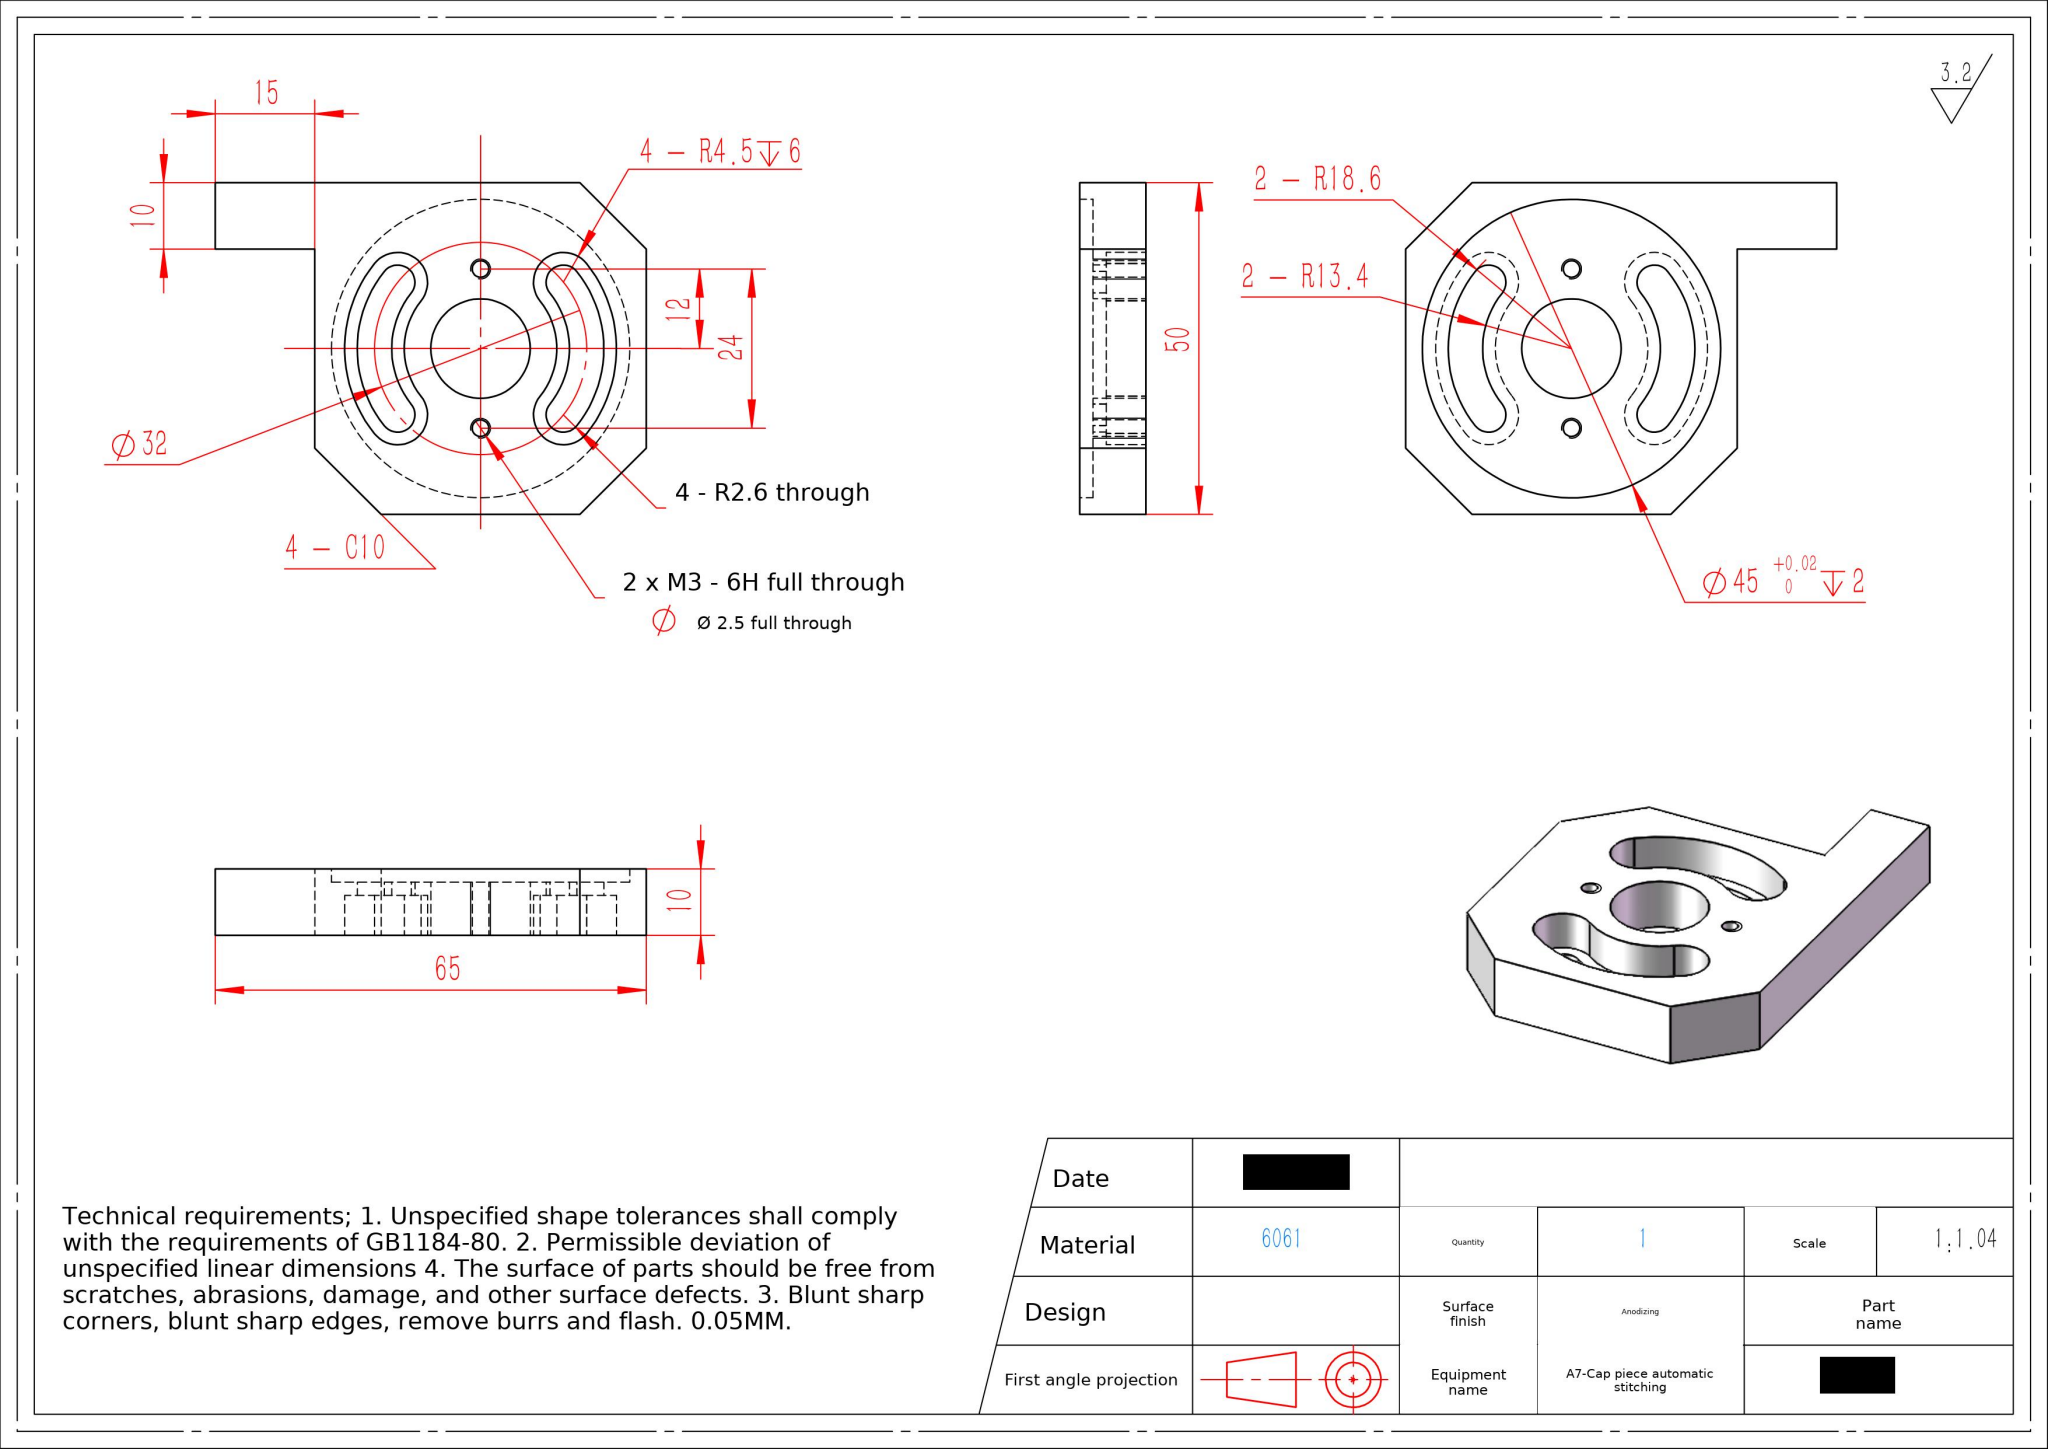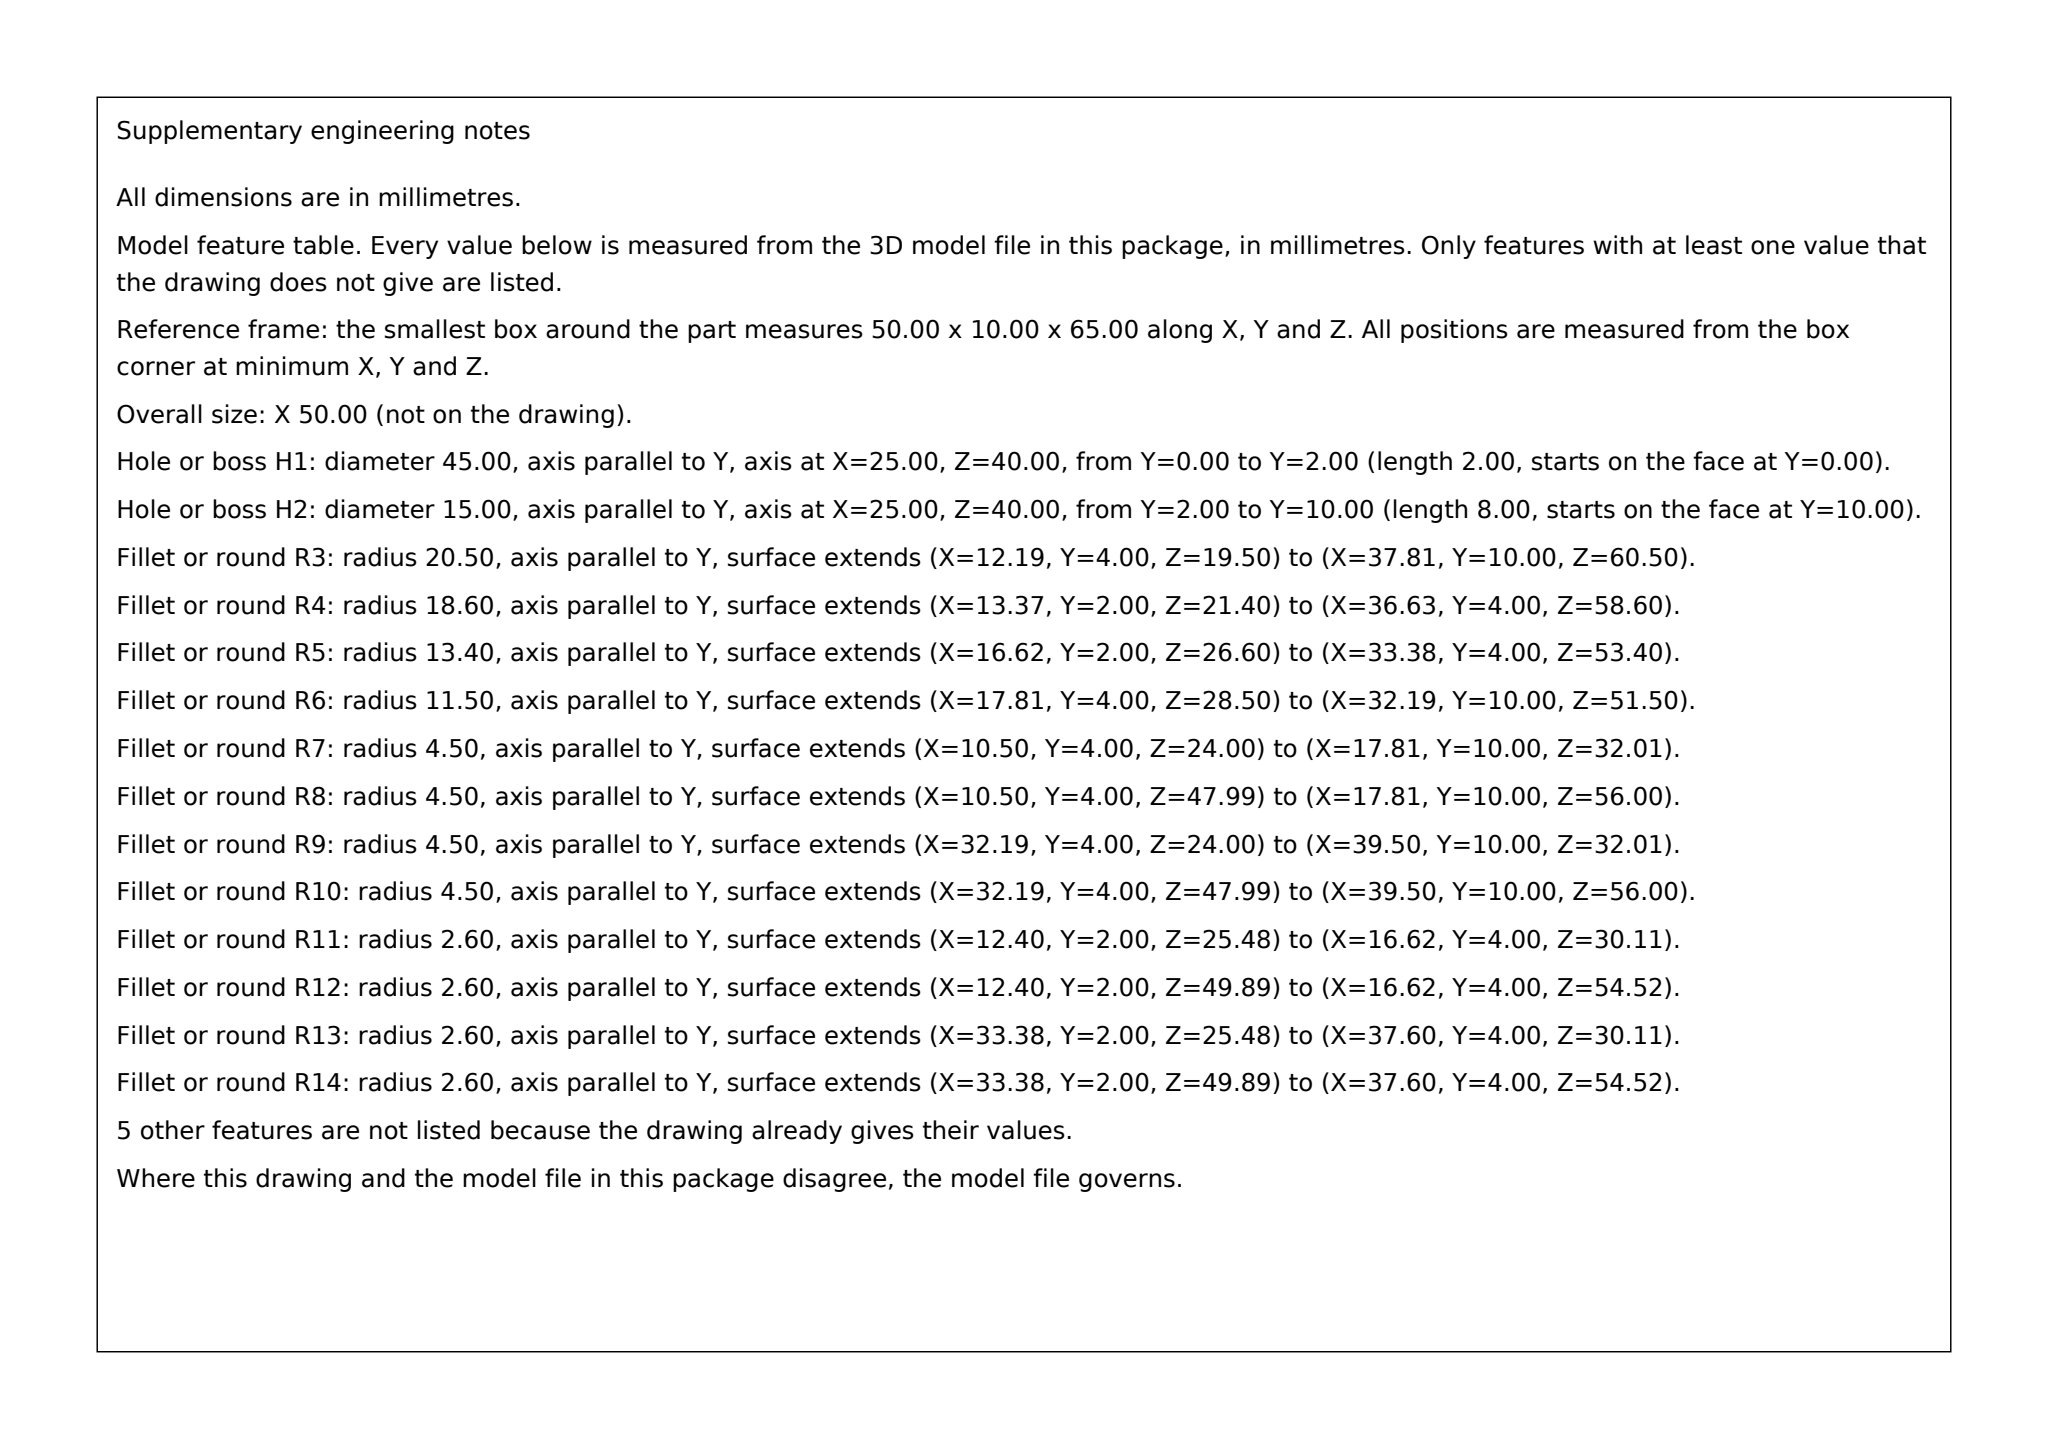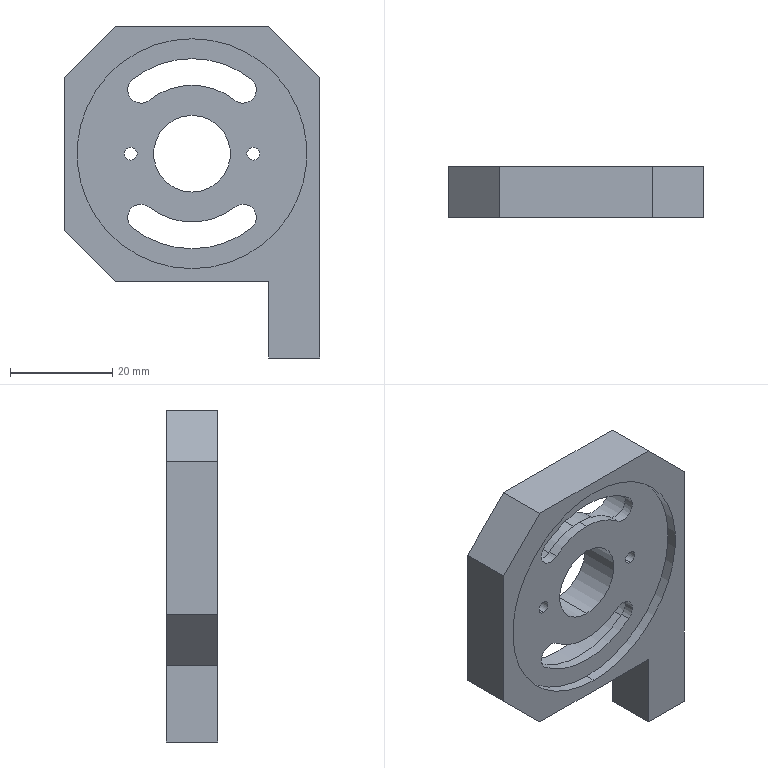Part | SolidWorks | mm | material 6061 | 1 solid | 46 faces | box 50 x 10 x 65 mm | volume 16696 mm3 | cylinder 32 | plane 14 | commonest cylinder face diameters 9 x6 5.2 x6 2.5 x4 41 x3 23 x3 37.2 x3 26.8 x3 45 x2
build123d program:
from build123d import *

# Parameters (mm, degrees)
SKETCH1_W           = 50
SKETCH1_H           = 50
BOSS_EXTRUDE1_DEPTH = 10
SKETCH2_R           = 7.5
CUT_EXTRUDE1_DEPTH  = 37.742
M3_TAPPED_HOLE1_D   = 2.5
SKETCH4_R           = 22.5
CUT_EXTRUDE2_DEPTH  = 2
CUT_EXTRUDE3_DEPTH  = 37.742
CUT_EXTRUDE4_DEPTH  = 6
SKETCH10_W          = 10
SKETCH10_H          = 10
BOSS_EXTRUDE2_DEPTH = 15
CHAMFER1_SIZE       = 10


with BuildPart() as part:
    # Sketch1 → Boss-Extrude1 (new body)
    with BuildSketch(Plane(origin=(0, 0, 0), x_dir=(1, 0, 0), z_dir=(0, 1, 0))):
        Rectangle(SKETCH1_W, SKETCH1_H)
    extrude(amount=BOSS_EXTRUDE1_DEPTH)

    # Sketch2 → Cut-Extrude1 (cut, through all)
    with BuildSketch(Plane(origin=(0, 10, 0), x_dir=(1, 0, 0), z_dir=(0, 1, 0))):
        with Locations(Location((0, 0, 0), (0, 0, 270))):
            Circle(SKETCH2_R)
    extrude(amount=-CUT_EXTRUDE1_DEPTH, mode=Mode.SUBTRACT)

    # M3 Tapped Hole1 (through all)
    with Locations(Plane(origin=(12, 10, 0), x_dir=(0, 0, 1), z_dir=(0, 1, 0))):
        with Locations((0, 0)):
            m3_tapped_hole1 = Hole(M3_TAPPED_HOLE1_D / 2)

    # Mirror1: M3 Tapped Hole1 across plane
    add(m3_tapped_hole1.mirror(Plane(origin=(0, 0, 0), x_dir=(0, 0, 1), z_dir=(1, 0, 0))), mode=Mode.SUBTRACT)

    # Sketch4 → Cut-Extrude2 (cut)
    with BuildSketch(Plane(origin=(0, 0, 0), x_dir=(-1, 0, 0), z_dir=(0, -1, 0))):
        with Locations(Location((0, 0, 0), (0, 0, 90))):
            Circle(SKETCH4_R)
    extrude(amount=-CUT_EXTRUDE2_DEPTH, mode=Mode.SUBTRACT)

    # Sketch5 → Cut-Extrude3 (cut, through all)
    with BuildSketch(Plane(origin=(0, 10, 0), x_dir=(1, 0, 0), z_dir=(0, 1, 0))):
        with BuildLine():
            ThreePointArc((-11.625, -14.52), (0, -18.6), (11.625, -14.52))
            ThreePointArc((11.625, -14.52), (12.03, -10.865), (8.375, -10.46))
            ThreePointArc((8.375, -10.46), (0, -13.4), (-8.375, -10.46))
            ThreePointArc((-8.375, -10.46), (-12.03, -10.865), (-11.625, -14.52))
        make_face()
    cut_extrude3 = extrude(amount=-CUT_EXTRUDE3_DEPTH, mode=Mode.SUBTRACT)

    # Sketch6 → Cut-Extrude4 (cut)
    with BuildSketch(Plane(origin=(0, 10, 0), x_dir=(1, 0, 0), z_dir=(0, 1, 0))):
        with BuildLine():
            ThreePointArc((-12.812, -16.003), (0, -20.5), (12.812, -16.003))
            ThreePointArc((12.812, -16.003), (13.513, -9.677), (7.188, -8.977))
            ThreePointArc((7.188, -8.977), (0, -11.5), (-7.188, -8.977))
            ThreePointArc((-7.188, -8.977), (-13.513, -9.677), (-12.812, -16.003))
        make_face()
    cut_extrude4 = extrude(amount=-CUT_EXTRUDE4_DEPTH, mode=Mode.SUBTRACT)

    # Mirror2: Cut-Extrude3, Cut-Extrude4 across plane
    add(cut_extrude3.mirror(Plane.XY), mode=Mode.SUBTRACT)
    add(cut_extrude4.mirror(Plane.XY), mode=Mode.SUBTRACT)

    # Sketch10 → Boss-Extrude2 (add)
    with BuildSketch(Plane(origin=(0, 0, -25), x_dir=(-1, 0, 0), z_dir=(0, 0, -1))):
        with Locations((-20, 5)):
            Rectangle(SKETCH10_W, SKETCH10_H)
    extrude(amount=BOSS_EXTRUDE2_DEPTH)

    # Chamfer1
    chamfer1_edges = [part.edges().sort_by_distance(p)[0] for p in [
        (25, 5, 25),
        (-25, 5, 25),
        (-25, 5, -25),
    ]]
    chamfer(chamfer1_edges, length=CHAMFER1_SIZE)


solid = part.part